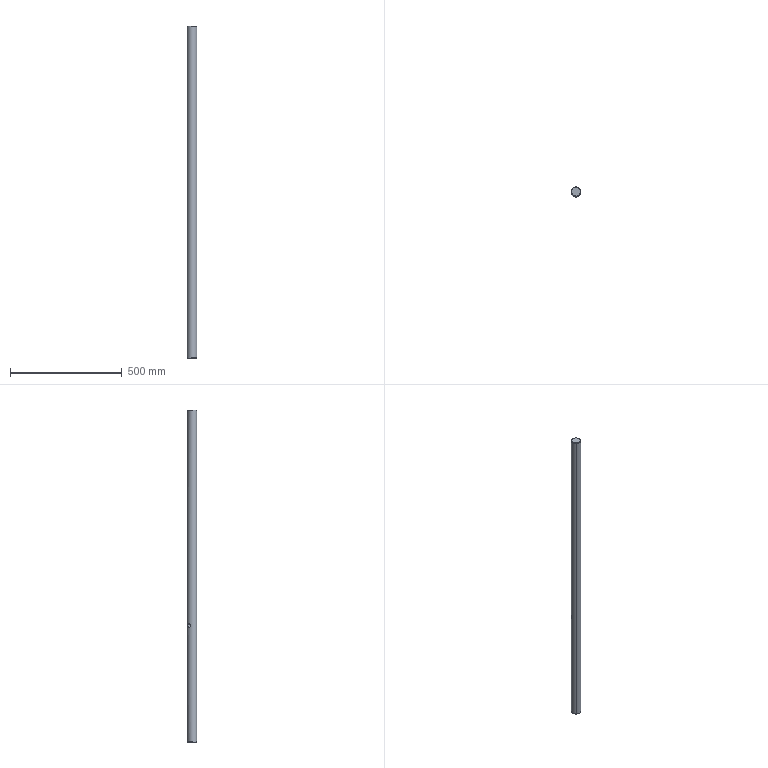Component | SolidWorks | Mandrel2-1 | 1 solid | 11 faces | box 43 x 43 x 1486.94 mm | volume 2152982 mm3 | cone 4 | cylinder 4 | plane 3 | commonest cylinder face diameters 16 x2 43 x2 | material 45
build123d program:
from build123d import *

# Parameters (mm, degrees)
SKETCH1_R           = 21.5
BOSS_EXTRUDE1_DEPTH = 997
SKETCH2_R           = 21.5
BOSS_EXTRUDE3_DEPTH = 489.94
SKETCH3_R           = 8
CUT_EXTRUDE1_DEPTH  = 539
CHAMFER1_SIZE       = 2


with BuildPart() as part:
    # Sketch1 → Boss-Extrude1 (new body)
    with BuildSketch(Plane.XY):
        with Locations((1397.317, -531.123)):
            Circle(SKETCH1_R)
    extrude(amount=BOSS_EXTRUDE1_DEPTH)

    # Sketch2 → Boss-Extrude3 (add)
    with BuildSketch(Plane.XY.offset(997)):
        with Locations((1397.317, -531.123)):
            Circle(SKETCH2_R)
    extrude(amount=BOSS_EXTRUDE3_DEPTH)

    # Sketch3 → Cut-Extrude1 (cut)
    with BuildSketch(Plane(origin=(0, 0, 0), x_dir=(1, 0, 0), z_dir=(0, 1, 0))):
        with Locations(Location((1397.317, -521.283, 0), (0, 0, 270))):
            Circle(SKETCH3_R)
    extrude(amount=-CUT_EXTRUDE1_DEPTH, mode=Mode.SUBTRACT)

    # Chamfer1
    chamfer1_edges = [part.edges().sort_by_distance(p)[0] for p in [
        (1375.817, -531.123, 0),
        (1375.817, -531.123, 1486.94),
    ]]
    chamfer(chamfer1_edges, length=CHAMFER1_SIZE)


solid = part.part

# Placed as in the assembly
solid = solid.moved(Location((206.204, -1339.515, -248.47), (0, 0, 51.912)))
STEP:
#1=COLOUR_RGB('',0.7922,0.8196,0.9333);
#2=FILL_AREA_STYLE_COLOUR('',#1);
#3=FILL_AREA_STYLE('',(#2));
#4=SURFACE_STYLE_FILL_AREA(#3);
#5=SURFACE_SIDE_STYLE('',(#4));
#6=SURFACE_STYLE_USAGE(.BOTH.,#5);
#7=PRESENTATION_STYLE_ASSIGNMENT((#6));
#8=CARTESIAN_POINT('',(58.985,-21.733,48.759));
#9=VERTEX_POINT('',#8);
#10=CARTESIAN_POINT('',(58.038,-22.942,48.759));
#11=VERTEX_POINT('',#10);
#12=CARTESIAN_POINT('',(58.512,-22.338,48.759));
#13=DIRECTION('',(0.,-0.,1.));
#14=DIRECTION('',(0.6169,0.7871,0.));
#15=AXIS2_PLACEMENT_3D('',#12,#13,#14);
#16=CIRCLE('',#15,0.7677);
#17=EDGE_CURVE('',#9,#11,#16,.T.);
#18=ORIENTED_EDGE('',*,*,#17,.F.);
#19=CARTESIAN_POINT('',(59.034,-21.671,48.68));
#20=VERTEX_POINT('',#19);
#21=CARTESIAN_POINT('',(58.985,-21.733,48.759));
#22=DIRECTION('',(0.4362,0.5565,-0.7071));
#23=VECTOR('',#22,39.37);
#24=LINE('',#21,#23);
#25=EDGE_CURVE('',#9,#20,#24,.T.);
#26=ORIENTED_EDGE('',*,*,#25,.T.);
#27=CARTESIAN_POINT('',(57.99,-23.004,48.68));
#28=VERTEX_POINT('',#27);
#29=CARTESIAN_POINT('',(58.512,-22.338,48.68));
#30=DIRECTION('',(-0.,0.,-1.));
#31=DIRECTION('',(0.6169,0.7871,0.));
#32=AXIS2_PLACEMENT_3D('',#29,#30,#31);
#33=CIRCLE('',#32,0.8465);
#34=EDGE_CURVE('',#28,#20,#33,.T.);
#35=ORIENTED_EDGE('',*,*,#34,.F.);
#36=CARTESIAN_POINT('',(58.038,-22.942,48.759));
#37=DIRECTION('',(-0.4362,-0.5565,-0.7071));
#38=VECTOR('',#37,39.37);
#39=LINE('',#36,#38);
#40=EDGE_CURVE('',#11,#28,#39,.T.);
#41=ORIENTED_EDGE('',*,*,#40,.F.);
#42=EDGE_LOOP('',(#18,#26,#35,#41));
#43=FACE_OUTER_BOUND('',#42,.T.);
#44=CARTESIAN_POINT('',(58.512,-22.338,48.759));
#45=DIRECTION('',(-0.,0.,-1.));
#46=DIRECTION('',(-0.6169,-0.7871,0.));
#47=AXIS2_PLACEMENT_3D('',#44,#45,#46);
#48=CONICAL_SURFACE('',#47,0.7677,0.7854);
#49=ADVANCED_FACE('',(#43),#48,.T.);
#50=CARTESIAN_POINT('',(58.038,-22.942,-9.782));
#51=VERTEX_POINT('',#50);
#52=CARTESIAN_POINT('',(58.985,-21.733,-9.782));
#53=VERTEX_POINT('',#52);
#54=CARTESIAN_POINT('',(58.512,-22.338,-9.782));
#55=DIRECTION('',(-0.,0.,-1.));
#56=DIRECTION('',(0.6169,0.7871,0.));
#57=AXIS2_PLACEMENT_3D('',#54,#55,#56);
#58=CIRCLE('',#57,0.7677);
#59=EDGE_CURVE('',#51,#53,#58,.T.);
#60=ORIENTED_EDGE('',*,*,#59,.F.);
#61=CARTESIAN_POINT('',(57.99,-23.004,-9.704));
#62=VERTEX_POINT('',#61);
#63=CARTESIAN_POINT('',(57.99,-23.004,-9.704));
#64=DIRECTION('',(-0.4362,-0.5565,0.7071));
#65=VECTOR('',#64,39.37);
#66=LINE('',#63,#65);
#67=EDGE_CURVE('',#51,#62,#66,.T.);
#68=ORIENTED_EDGE('',*,*,#67,.T.);
#69=CARTESIAN_POINT('',(59.034,-21.671,-9.704));
#70=VERTEX_POINT('',#69);
#71=CARTESIAN_POINT('',(58.512,-22.338,-9.704));
#72=DIRECTION('',(0.,-0.,1.));
#73=DIRECTION('',(0.6169,0.7871,0.));
#74=AXIS2_PLACEMENT_3D('',#71,#72,#73);
#75=CIRCLE('',#74,0.8465);
#76=EDGE_CURVE('',#70,#62,#75,.T.);
#77=ORIENTED_EDGE('',*,*,#76,.F.);
#78=CARTESIAN_POINT('',(59.034,-21.671,-9.704));
#79=DIRECTION('',(0.4362,0.5565,0.7071));
#80=VECTOR('',#79,39.37);
#81=LINE('',#78,#80);
#82=EDGE_CURVE('',#53,#70,#81,.T.);
#83=ORIENTED_EDGE('',*,*,#82,.F.);
#84=EDGE_LOOP('',(#60,#68,#77,#83));
#85=FACE_OUTER_BOUND('',#84,.T.);
#86=CARTESIAN_POINT('',(58.512,-22.338,-9.704));
#87=DIRECTION('',(0.,-0.,1.));
#88=DIRECTION('',(0.6169,0.7871,0.));
#89=AXIS2_PLACEMENT_3D('',#86,#87,#88);
#90=CONICAL_SURFACE('',#89,0.8465,0.7854);
#91=ADVANCED_FACE('',(#85),#90,.T.);
#92=CARTESIAN_POINT('',(58.756,-22.529,10.426));
#93=VERTEX_POINT('',#92);
#94=CARTESIAN_POINT('',(58.756,-22.529,11.056));
#95=VERTEX_POINT('',#94);
#96=CARTESIAN_POINT('',(58.756,-22.529,10.741));
#97=DIRECTION('',(-0.7871,0.6169,0.));
#98=DIRECTION('',(0.,0.,1.));
#99=AXIS2_PLACEMENT_3D('',#96,#97,#98);
#100=CIRCLE('',#99,0.315);
#101=EDGE_CURVE('',#93,#95,#100,.T.);
#102=ORIENTED_EDGE('',*,*,#101,.F.);
#103=CARTESIAN_POINT('',(57.846,-21.815,10.426));
#104=VERTEX_POINT('',#103);
#105=CARTESIAN_POINT('',(58.756,-22.529,10.426));
#106=DIRECTION('',(-0.7871,0.6169,0.));
#107=VECTOR('',#106,39.37);
#108=LINE('',#105,#107);
#109=EDGE_CURVE('',#93,#104,#108,.T.);
#110=ORIENTED_EDGE('',*,*,#109,.T.);
#111=CARTESIAN_POINT('',(57.846,-21.815,11.056));
#112=VERTEX_POINT('',#111);
#113=CARTESIAN_POINT('',(57.846,-21.815,11.056));
#114=CARTESIAN_POINT('',(57.833,-21.832,11.056));
#115=CARTESIAN_POINT('',(57.821,-21.849,11.054));
#116=CARTESIAN_POINT('',(57.804,-21.874,11.047));
#117=CARTESIAN_POINT('',(57.798,-21.882,11.045));
#118=CARTESIAN_POINT('',(57.788,-21.899,11.039));
#119=CARTESIAN_POINT('',(57.782,-21.908,11.035));
#120=CARTESIAN_POINT('',(57.768,-21.933,11.023));
#121=CARTESIAN_POINT('',(57.76,-21.949,11.014));
#122=CARTESIAN_POINT('',(57.748,-21.973,10.997));
#123=CARTESIAN_POINT('',(57.744,-21.98,10.99));
#124=CARTESIAN_POINT('',(57.738,-21.995,10.977));
#125=CARTESIAN_POINT('',(57.735,-22.002,10.97));
#126=CARTESIAN_POINT('',(57.726,-22.023,10.949));
#127=CARTESIAN_POINT('',(57.721,-22.036,10.933));
#128=CARTESIAN_POINT('',(57.713,-22.058,10.899));
#129=CARTESIAN_POINT('',(57.709,-22.068,10.881));
#130=CARTESIAN_POINT('',(57.705,-22.08,10.852));
#131=CARTESIAN_POINT('',(57.704,-22.084,10.843));
#132=CARTESIAN_POINT('',(57.702,-22.09,10.823));
#133=CARTESIAN_POINT('',(57.702,-22.092,10.813));
#134=CARTESIAN_POINT('',(57.7,-22.099,10.782));
#135=CARTESIAN_POINT('',(57.699,-22.101,10.762));
#136=CARTESIAN_POINT('',(57.699,-22.101,10.72));
#137=CARTESIAN_POINT('',(57.7,-22.099,10.699));
#138=CARTESIAN_POINT('',(57.702,-22.09,10.658));
#139=CARTESIAN_POINT('',(57.704,-22.084,10.639));
#140=CARTESIAN_POINT('',(57.709,-22.068,10.6));
#141=CARTESIAN_POINT('',(57.713,-22.058,10.582));
#142=CARTESIAN_POINT('',(57.719,-22.041,10.557));
#143=CARTESIAN_POINT('',(57.721,-22.035,10.549));
#144=CARTESIAN_POINT('',(57.726,-22.023,10.533));
#145=CARTESIAN_POINT('',(57.729,-22.016,10.525));
#146=CARTESIAN_POINT('',(57.738,-21.995,10.503));
#147=CARTESIAN_POINT('',(57.744,-21.981,10.49));
#148=CARTESIAN_POINT('',(57.756,-21.957,10.473));
#149=CARTESIAN_POINT('',(57.76,-21.949,10.468));
#150=CARTESIAN_POINT('',(57.768,-21.933,10.458));
#151=CARTESIAN_POINT('',(57.773,-21.924,10.454));
#152=CARTESIAN_POINT('',(57.787,-21.9,10.442));
#153=CARTESIAN_POINT('',(57.798,-21.883,10.436));
#154=CARTESIAN_POINT('',(57.815,-21.857,10.43));
#155=CARTESIAN_POINT('',(57.821,-21.849,10.428));
#156=CARTESIAN_POINT('',(57.833,-21.832,10.426));
#157=CARTESIAN_POINT('',(57.839,-21.824,10.426));
#158=CARTESIAN_POINT('',(57.846,-21.815,10.426));
#159=B_SPLINE_CURVE_WITH_KNOTS('',3,(#113,#114,#115,#116,#117,#118,#119,#120,#121,#122,#123,#124,#125,#126,#127,#128,#129,#130,#131,#132,#133,#134,#135,#136,#137,#138,#139,#140,#141,#142,#143,#144,#145,#146,#147,#148,#149,#150,#151,#152,#153,#154,#155,#156,#157,#158),.UNSPECIFIED.,.F.,.F.,(4,2,2,2,2,2,2,2,2,2,2,2,2,2,2,2,2,2,2,2,2,2,4),(0.,0.001578,0.002366,0.003155,0.004733,0.005521,0.00631,0.007888,0.009465,0.01025,0.01104,0.01262,0.0142,0.01578,0.01735,0.01814,0.01893,0.02051,0.0213,0.02209,0.02366,0.02445,0.02524),.UNSPECIFIED.);
#160=EDGE_CURVE('',#112,#104,#159,.T.);
#161=ORIENTED_EDGE('',*,*,#160,.F.);
#162=CARTESIAN_POINT('',(58.756,-22.529,11.056));
#163=DIRECTION('',(-0.7871,0.6169,0.));
#164=VECTOR('',#163,39.37);
#165=LINE('',#162,#164);
#166=EDGE_CURVE('',#95,#112,#165,.T.);
#167=ORIENTED_EDGE('',*,*,#166,.F.);
#168=EDGE_LOOP('',(#102,#110,#161,#167));
#169=FACE_OUTER_BOUND('',#168,.T.);
#170=CARTESIAN_POINT('',(58.756,-22.529,10.741));
#171=DIRECTION('',(-0.7871,0.6169,0.));
#172=DIRECTION('',(0.,0.,1.));
#173=AXIS2_PLACEMENT_3D('',#170,#171,#172);
#174=CYLINDRICAL_SURFACE('',#173,0.315);
#175=ADVANCED_FACE('',(#169),#174,.F.);
#176=ORIENTED_EDGE('',*,*,#160,.T.);
#177=CARTESIAN_POINT('',(57.846,-21.815,10.426));
#178=CARTESIAN_POINT('',(57.852,-21.807,10.426));
#179=CARTESIAN_POINT('',(57.859,-21.799,10.426));
#180=CARTESIAN_POINT('',(57.872,-21.783,10.428));
#181=CARTESIAN_POINT('',(57.879,-21.776,10.43));
#182=CARTESIAN_POINT('',(57.899,-21.753,10.436));
#183=CARTESIAN_POINT('',(57.913,-21.739,10.442));
#184=CARTESIAN_POINT('',(57.934,-21.719,10.454));
#185=CARTESIAN_POINT('',(57.941,-21.712,10.458));
#186=CARTESIAN_POINT('',(57.955,-21.7,10.468));
#187=CARTESIAN_POINT('',(57.962,-21.694,10.473));
#188=CARTESIAN_POINT('',(57.982,-21.678,10.491));
#189=CARTESIAN_POINT('',(57.994,-21.668,10.504));
#190=CARTESIAN_POINT('',(58.019,-21.649,10.533));
#191=CARTESIAN_POINT('',(58.03,-21.642,10.548));
#192=CARTESIAN_POINT('',(58.045,-21.632,10.574));
#193=CARTESIAN_POINT('',(58.049,-21.629,10.583));
#194=CARTESIAN_POINT('',(58.058,-21.623,10.601));
#195=CARTESIAN_POINT('',(58.062,-21.621,10.61));
#196=CARTESIAN_POINT('',(58.073,-21.614,10.639));
#197=CARTESIAN_POINT('',(58.078,-21.611,10.658));
#198=CARTESIAN_POINT('',(58.086,-21.606,10.699));
#199=CARTESIAN_POINT('',(58.088,-21.605,10.72));
#200=CARTESIAN_POINT('',(58.088,-21.605,10.762));
#201=CARTESIAN_POINT('',(58.086,-21.606,10.782));
#202=CARTESIAN_POINT('',(58.08,-21.61,10.813));
#203=CARTESIAN_POINT('',(58.078,-21.611,10.823));
#204=CARTESIAN_POINT('',(58.072,-21.614,10.843));
#205=CARTESIAN_POINT('',(58.069,-21.616,10.852));
#206=CARTESIAN_POINT('',(58.062,-21.621,10.871));
#207=CARTESIAN_POINT('',(58.058,-21.623,10.881));
#208=CARTESIAN_POINT('',(58.049,-21.629,10.899));
#209=CARTESIAN_POINT('',(58.044,-21.632,10.908));
#210=CARTESIAN_POINT('',(58.03,-21.642,10.933));
#211=CARTESIAN_POINT('',(58.018,-21.65,10.949));
#212=CARTESIAN_POINT('',(57.994,-21.668,10.978));
#213=CARTESIAN_POINT('',(57.981,-21.678,10.991));
#214=CARTESIAN_POINT('',(57.955,-21.7,11.014));
#215=CARTESIAN_POINT('',(57.941,-21.712,11.023));
#216=CARTESIAN_POINT('',(57.92,-21.732,11.035));
#217=CARTESIAN_POINT('',(57.913,-21.739,11.039));
#218=CARTESIAN_POINT('',(57.899,-21.753,11.045));
#219=CARTESIAN_POINT('',(57.892,-21.761,11.047));
#220=CARTESIAN_POINT('',(57.872,-21.783,11.054));
#221=CARTESIAN_POINT('',(57.859,-21.799,11.056));
#222=CARTESIAN_POINT('',(57.846,-21.815,11.056));
#223=B_SPLINE_CURVE_WITH_KNOTS('',3,(#177,#178,#179,#180,#181,#182,#183,#184,#185,#186,#187,#188,#189,#190,#191,#192,#193,#194,#195,#196,#197,#198,#199,#200,#201,#202,#203,#204,#205,#206,#207,#208,#209,#210,#211,#212,#213,#214,#215,#216,#217,#218,#219,#220,#221,#222),.UNSPECIFIED.,.F.,.F.,(4,2,2,2,2,2,2,2,2,2,2,2,2,2,2,2,2,2,2,2,2,2,4),(0.02524,0.02603,0.02682,0.0284,0.02918,0.02997,0.03155,0.03313,0.03392,0.0347,0.03628,0.03786,0.03944,0.04022,0.04101,0.0418,0.04259,0.04417,0.04574,0.04732,0.04811,0.0489,0.05048),.UNSPECIFIED.);
#224=EDGE_CURVE('',#104,#112,#223,.T.);
#225=ORIENTED_EDGE('',*,*,#224,.T.);
#226=EDGE_LOOP('',(#176,#225));
#227=FACE_BOUND('',#226,.T.);
#228=ORIENTED_EDGE('',*,*,#34,.T.);
#229=CARTESIAN_POINT('',(59.034,-21.671,29.47));
#230=DIRECTION('',(-0.,0.,-1.));
#231=VECTOR('',#230,39.37);
#232=LINE('',#229,#231);
#233=EDGE_CURVE('',#20,#70,#232,.T.);
#234=ORIENTED_EDGE('',*,*,#233,.T.);
#235=ORIENTED_EDGE('',*,*,#76,.T.);
#236=CARTESIAN_POINT('',(57.99,-23.004,29.47));
#237=DIRECTION('',(-0.,0.,-1.));
#238=VECTOR('',#237,39.37);
#239=LINE('',#236,#238);
#240=EDGE_CURVE('',#28,#62,#239,.T.);
#241=ORIENTED_EDGE('',*,*,#240,.F.);
#242=EDGE_LOOP('',(#228,#234,#235,#241));
#243=FACE_OUTER_BOUND('',#242,.T.);
#244=CARTESIAN_POINT('',(58.512,-22.338,29.47));
#245=DIRECTION('',(-0.,0.,-1.));
#246=DIRECTION('',(-0.6169,-0.7871,0.));
#247=AXIS2_PLACEMENT_3D('',#244,#245,#246);
#248=CYLINDRICAL_SURFACE('',#247,0.8465);
#249=ADVANCED_FACE('',(#227,#243),#248,.T.);
#250=ORIENTED_EDGE('',*,*,#233,.F.);
#251=CARTESIAN_POINT('',(58.512,-22.338,48.68));
#252=DIRECTION('',(-0.,0.,-1.));
#253=DIRECTION('',(0.6169,0.7871,0.));
#254=AXIS2_PLACEMENT_3D('',#251,#252,#253);
#255=CIRCLE('',#254,0.8465);
#256=EDGE_CURVE('',#20,#28,#255,.T.);
#257=ORIENTED_EDGE('',*,*,#256,.T.);
#258=ORIENTED_EDGE('',*,*,#240,.T.);
#259=CARTESIAN_POINT('',(58.512,-22.338,-9.704));
#260=DIRECTION('',(0.,-0.,1.));
#261=DIRECTION('',(0.6169,0.7871,0.));
#262=AXIS2_PLACEMENT_3D('',#259,#260,#261);
#263=CIRCLE('',#262,0.8465);
#264=EDGE_CURVE('',#62,#70,#263,.T.);
#265=ORIENTED_EDGE('',*,*,#264,.T.);
#266=EDGE_LOOP('',(#250,#257,#258,#265));
#267=FACE_OUTER_BOUND('',#266,.T.);
#268=CARTESIAN_POINT('',(58.512,-22.338,29.47));
#269=DIRECTION('',(-0.,0.,-1.));
#270=DIRECTION('',(-0.6169,-0.7871,0.));
#271=AXIS2_PLACEMENT_3D('',#268,#269,#270);
#272=CYLINDRICAL_SURFACE('',#271,0.8465);
#273=ADVANCED_FACE('',(#267),#272,.T.);
#274=CARTESIAN_POINT('',(58.512,-22.338,-9.782));
#275=DIRECTION('',(-0.,0.,-1.));
#276=DIRECTION('',(0.6169,0.7871,0.));
#277=AXIS2_PLACEMENT_3D('',#274,#275,#276);
#278=CIRCLE('',#277,0.7677);
#279=EDGE_CURVE('',#53,#51,#278,.T.);
#280=ORIENTED_EDGE('',*,*,#279,.T.);
#281=ORIENTED_EDGE('',*,*,#59,.T.);
#282=EDGE_LOOP('',(#280,#281));
#283=FACE_OUTER_BOUND('',#282,.T.);
#284=CARTESIAN_POINT('',(58.512,-22.338,-9.782));
#285=DIRECTION('',(0.,-0.,1.));
#286=DIRECTION('',(0.6169,0.7871,0.));
#287=AXIS2_PLACEMENT_3D('',#284,#285,#286);
#288=PLANE('',#287);
#289=ADVANCED_FACE('',(#283),#288,.F.);
#290=CARTESIAN_POINT('',(58.512,-22.338,48.759));
#291=DIRECTION('',(0.,-0.,1.));
#292=DIRECTION('',(0.6169,0.7871,0.));
#293=AXIS2_PLACEMENT_3D('',#290,#291,#292);
#294=CIRCLE('',#293,0.7677);
#295=EDGE_CURVE('',#11,#9,#294,.T.);
#296=ORIENTED_EDGE('',*,*,#295,.T.);
#297=ORIENTED_EDGE('',*,*,#17,.T.);
#298=EDGE_LOOP('',(#296,#297));
#299=FACE_OUTER_BOUND('',#298,.T.);
#300=CARTESIAN_POINT('',(58.512,-22.338,48.759));
#301=DIRECTION('',(0.,-0.,1.));
#302=DIRECTION('',(0.6169,0.7871,0.));
#303=AXIS2_PLACEMENT_3D('',#300,#301,#302);
#304=PLANE('',#303);
#305=ADVANCED_FACE('',(#299),#304,.T.);
#306=ORIENTED_EDGE('',*,*,#109,.F.);
#307=CARTESIAN_POINT('',(58.756,-22.529,10.741));
#308=DIRECTION('',(-0.7871,0.6169,0.));
#309=DIRECTION('',(0.,0.,1.));
#310=AXIS2_PLACEMENT_3D('',#307,#308,#309);
#311=CIRCLE('',#310,0.315);
#312=EDGE_CURVE('',#95,#93,#311,.T.);
#313=ORIENTED_EDGE('',*,*,#312,.F.);
#314=ORIENTED_EDGE('',*,*,#166,.T.);
#315=ORIENTED_EDGE('',*,*,#224,.F.);
#316=EDGE_LOOP('',(#306,#313,#314,#315));
#317=FACE_OUTER_BOUND('',#316,.T.);
#318=CARTESIAN_POINT('',(58.756,-22.529,10.741));
#319=DIRECTION('',(-0.7871,0.6169,0.));
#320=DIRECTION('',(0.,0.,1.));
#321=AXIS2_PLACEMENT_3D('',#318,#319,#320);
#322=CYLINDRICAL_SURFACE('',#321,0.315);
#323=ADVANCED_FACE('',(#317),#322,.F.);
#324=ORIENTED_EDGE('',*,*,#312,.T.);
#325=ORIENTED_EDGE('',*,*,#101,.T.);
#326=EDGE_LOOP('',(#324,#325));
#327=FACE_OUTER_BOUND('',#326,.T.);
#328=CARTESIAN_POINT('',(58.756,-22.529,10.741));
#329=DIRECTION('',(-0.7871,0.6169,0.));
#330=DIRECTION('',(0.,-0.,1.));
#331=AXIS2_PLACEMENT_3D('',#328,#329,#330);
#332=PLANE('',#331);
#333=ADVANCED_FACE('',(#327),#332,.T.);
#334=ORIENTED_EDGE('',*,*,#67,.F.);
#335=ORIENTED_EDGE('',*,*,#279,.F.);
#336=ORIENTED_EDGE('',*,*,#82,.T.);
#337=ORIENTED_EDGE('',*,*,#264,.F.);
#338=EDGE_LOOP('',(#334,#335,#336,#337));
#339=FACE_OUTER_BOUND('',#338,.T.);
#340=CARTESIAN_POINT('',(58.512,-22.338,-9.704));
#341=DIRECTION('',(0.,-0.,1.));
#342=DIRECTION('',(0.6169,0.7871,0.));
#343=AXIS2_PLACEMENT_3D('',#340,#341,#342);
#344=CONICAL_SURFACE('',#343,0.8465,0.7854);
#345=ADVANCED_FACE('',(#339),#344,.T.);
#346=ORIENTED_EDGE('',*,*,#25,.F.);
#347=ORIENTED_EDGE('',*,*,#295,.F.);
#348=ORIENTED_EDGE('',*,*,#40,.T.);
#349=ORIENTED_EDGE('',*,*,#256,.F.);
#350=EDGE_LOOP('',(#346,#347,#348,#349));
#351=FACE_OUTER_BOUND('',#350,.T.);
#352=CARTESIAN_POINT('',(58.512,-22.338,48.759));
#353=DIRECTION('',(-0.,0.,-1.));
#354=DIRECTION('',(-0.6169,-0.7871,0.));
#355=AXIS2_PLACEMENT_3D('',#352,#353,#354);
#356=CONICAL_SURFACE('',#355,0.7677,0.7854);
#357=ADVANCED_FACE('',(#351),#356,.T.);
#358=CLOSED_SHELL('',(#49,#91,#175,#249,#273,#289,#305,#323,#333,#345,#357));
#359=MANIFOLD_SOLID_BREP('',#358);
#360=STYLED_ITEM('',(#7),#359);
#361=PRESENTATION_LAYER_ASSIGNMENT('','',(#360));
#362=(LENGTH_UNIT()NAMED_UNIT(*)SI_UNIT($,.METRE.));
#363=LENGTH_MEASURE_WITH_UNIT(LENGTH_MEASURE(0.0254),#362);
#364=DIMENSIONAL_EXPONENTS(1.,0.,0.,0.,0.,0.,0.);
#365=(CONVERSION_BASED_UNIT('',#363)LENGTH_UNIT()NAMED_UNIT(#364));
#366=UNCERTAINTY_MEASURE_WITH_UNIT(LENGTH_MEASURE(0.00001),#365,'','');
#367=(NAMED_UNIT(*)PLANE_ANGLE_UNIT()SI_UNIT($,.RADIAN.));
#368=(NAMED_UNIT(*)SI_UNIT($,.STERADIAN.)SOLID_ANGLE_UNIT());
#369=(GEOMETRIC_REPRESENTATION_CONTEXT(3)GLOBAL_UNCERTAINTY_ASSIGNED_CONTEXT((#366))GLOBAL_UNIT_ASSIGNED_CONTEXT((#365,#367,#368))REPRESENTATION_CONTEXT('',''));
#370=MECHANICAL_DESIGN_GEOMETRIC_PRESENTATION_REPRESENTATION('',(#360),#369);
#371=CARTESIAN_POINT('',(0.,0.,0.));
#372=DIRECTION('',(0.,0.,1.));
#373=DIRECTION('',(1.,0.,0.));
#374=AXIS2_PLACEMENT_3D('',#371,#372,#373);
#375=(LENGTH_UNIT()NAMED_UNIT(*)SI_UNIT($,.METRE.));
#376=LENGTH_MEASURE_WITH_UNIT(LENGTH_MEASURE(0.0254),#375);
#377=DIMENSIONAL_EXPONENTS(1.,0.,0.,0.,0.,0.,0.);
#378=(CONVERSION_BASED_UNIT('',#376)LENGTH_UNIT()NAMED_UNIT(#377));
#379=UNCERTAINTY_MEASURE_WITH_UNIT(LENGTH_MEASURE(0.00001),#378,'','');
#380=(NAMED_UNIT(*)PLANE_ANGLE_UNIT()SI_UNIT($,.RADIAN.));
#381=(NAMED_UNIT(*)SI_UNIT($,.STERADIAN.)SOLID_ANGLE_UNIT());
#382=(GEOMETRIC_REPRESENTATION_CONTEXT(3)GLOBAL_UNCERTAINTY_ASSIGNED_CONTEXT((#379))GLOBAL_UNIT_ASSIGNED_CONTEXT((#378,#380,#381))REPRESENTATION_CONTEXT('',''));
#383=ADVANCED_BREP_SHAPE_REPRESENTATION('',(#359,#374),#382);